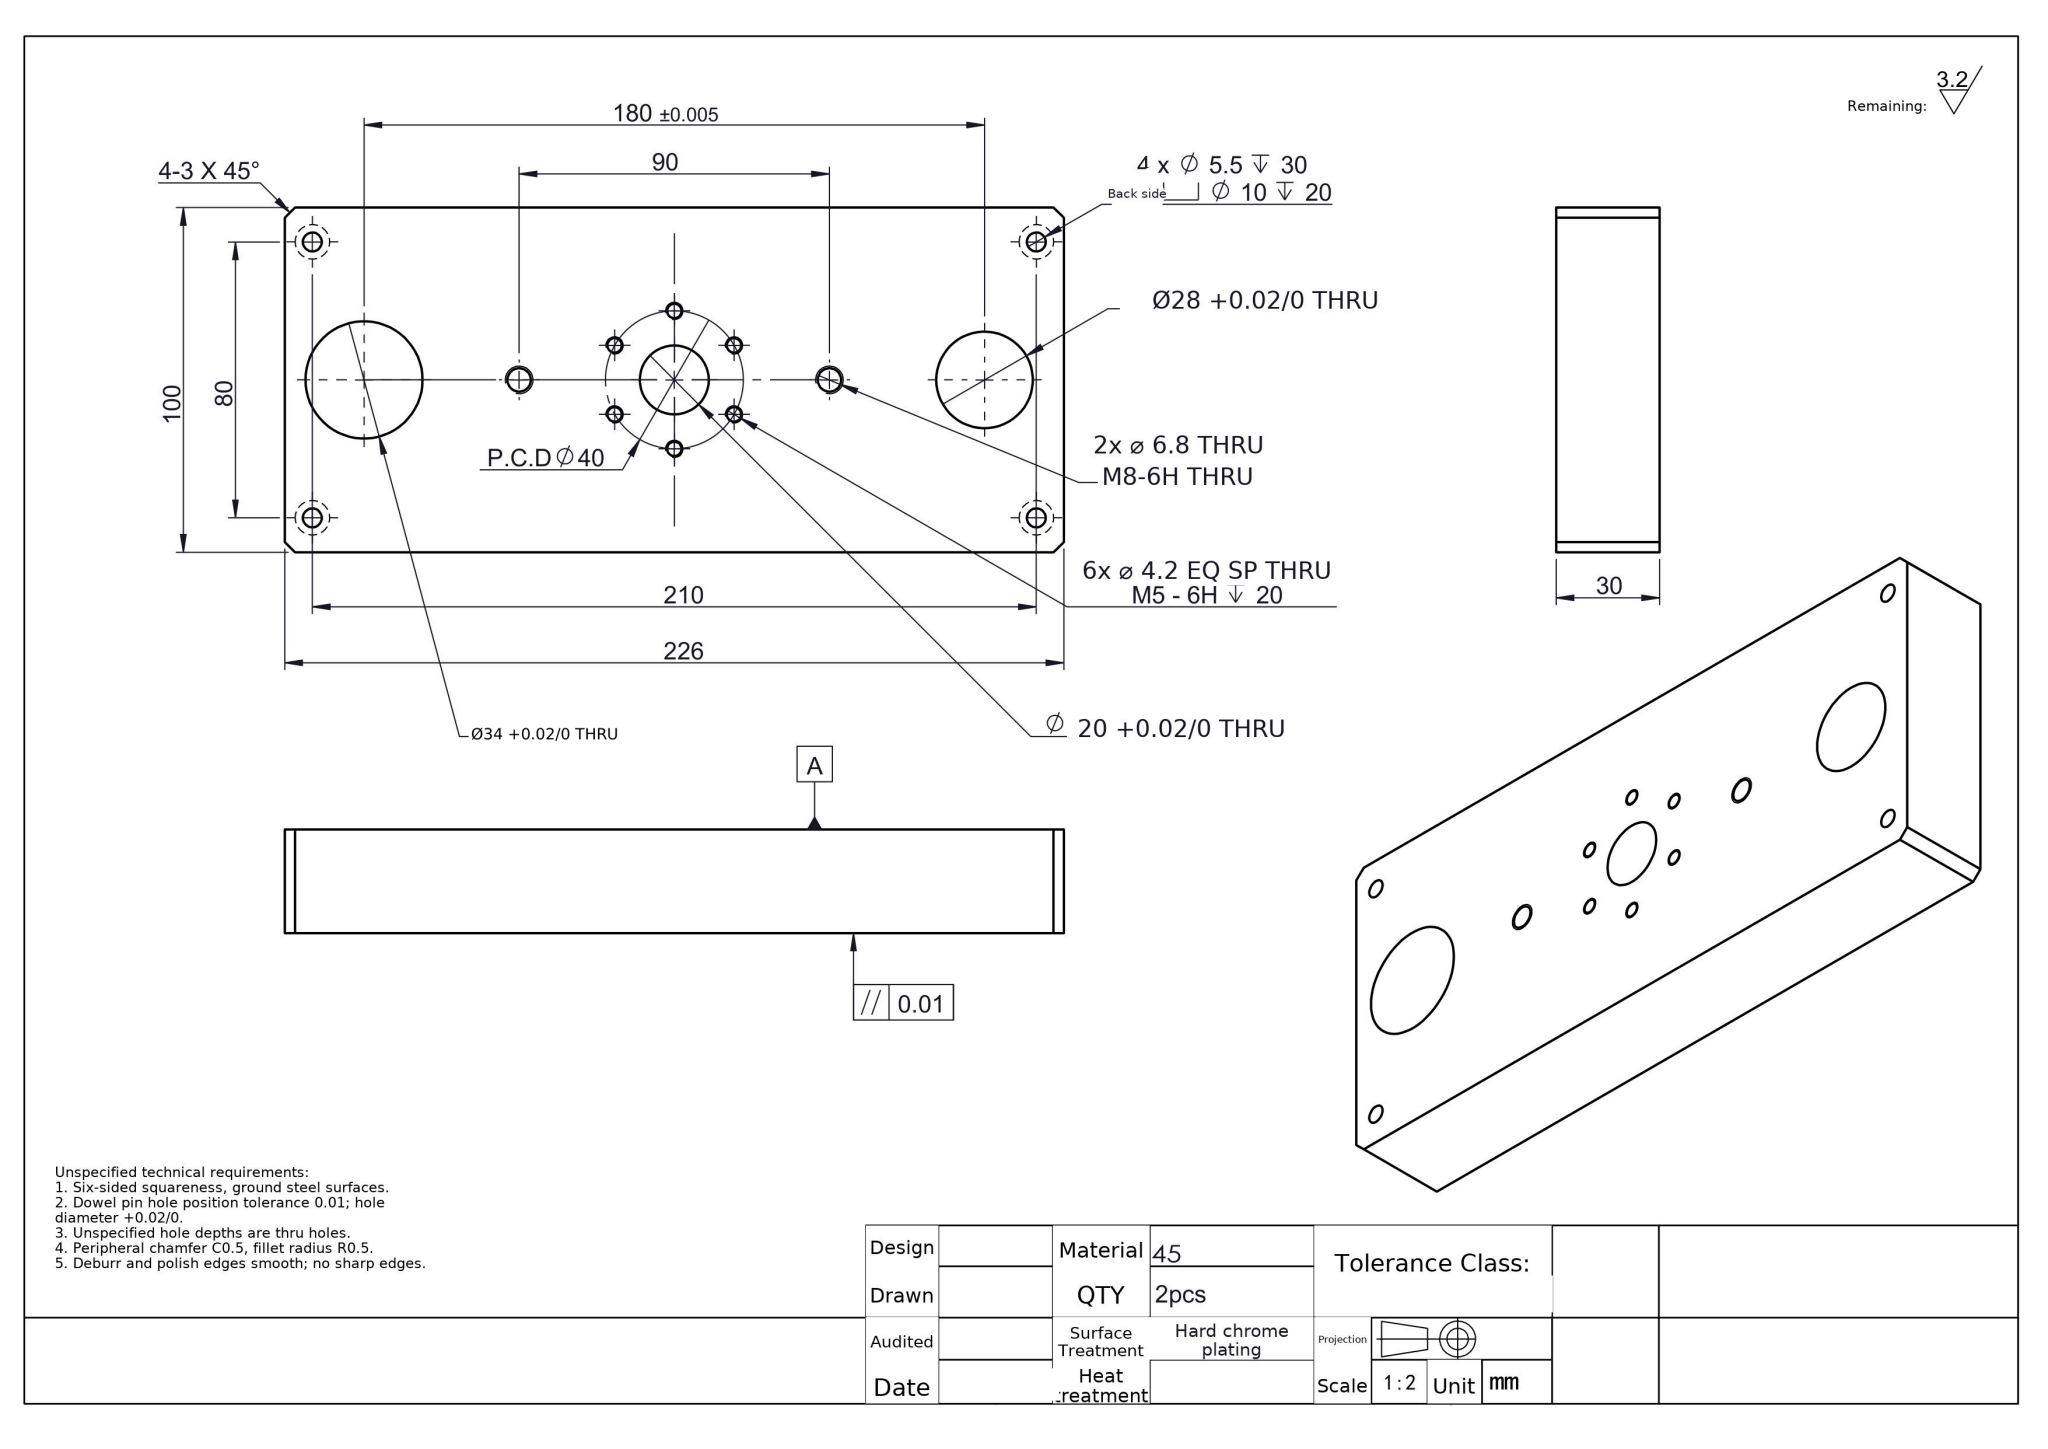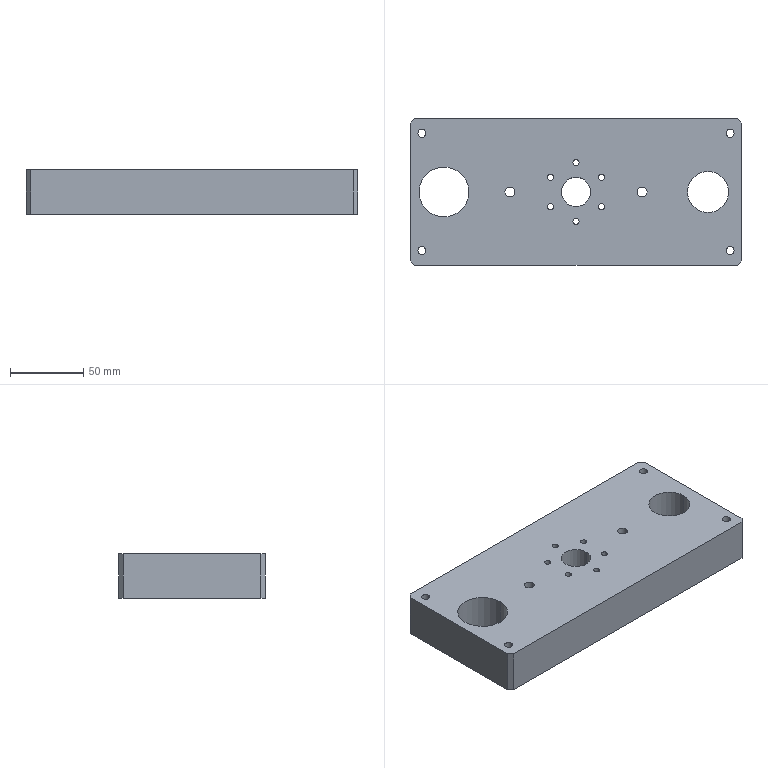Part | NX | mm | 1 solid | 52 faces | box 226 x 100 x 30 mm | volume 610419 mm3 | cylinder 38 | plane 14 | commonest cylinder face diameters 4.2 x12 10 x8 5.5 x8 6.8 x4 28 x2 34 x2 20 x2